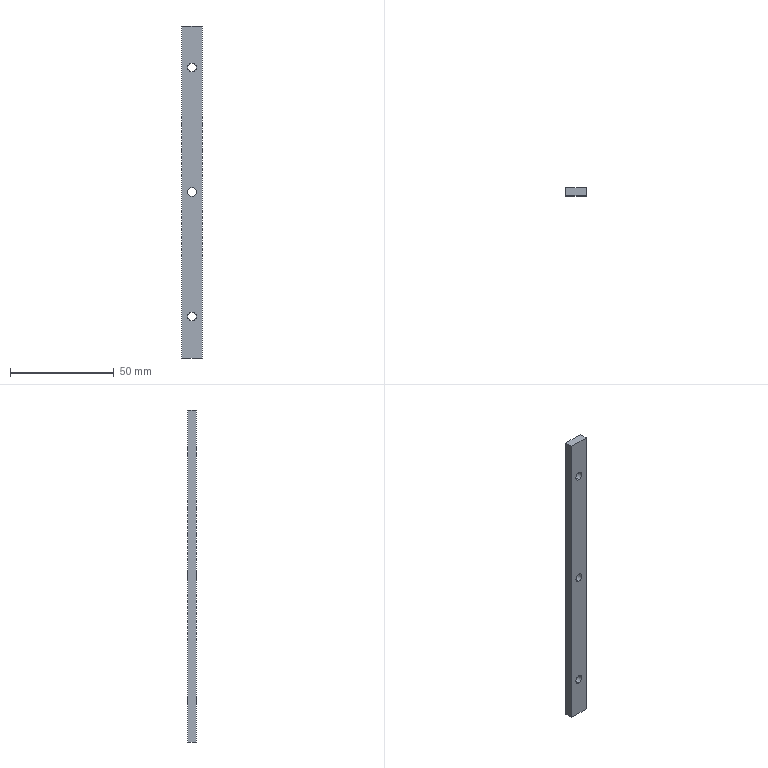Component | SolidWorks | Cover1-6XG1-1 | 1 solid | 12 faces | box 10 x 4 x 160 mm | volume 6234 mm3 | cylinder 6 | plane 6 | commonest cylinder face diameters 4.2 x6
build123d program:
from build123d import *

# Parameters (mm, degrees)
SKETCH1_W           = 160
SKETCH1_H           = 10
BOSS_EXTRUDE1_DEPTH = 4
M5_TAPPED_HOLE1_D   = 4.2


with BuildPart() as part:
    # Sketch1 → Boss-Extrude1 (new body)
    with BuildSketch(Plane.XY):
        Rectangle(SKETCH1_W, SKETCH1_H)
    extrude(amount=BOSS_EXTRUDE1_DEPTH)

    # M5 Tapped Hole1 (through all)
    with Locations(Plane.XY.offset(4)):
        with Locations((-60, 0), (0, 0), (60, 0)):
            Hole(M5_TAPPED_HOLE1_D / 2)


solid = part.part

# Placed as in the assembly
solid = solid.moved(Location((93.5, -154.8, 130), (90, 0, 90)))
STEP:
#1=CARTESIAN_POINT('',(3.681,-6.094,7.563));
#2=VERTEX_POINT('',#1);
#3=CARTESIAN_POINT('',(3.681,-6.094,7.398));
#4=VERTEX_POINT('',#3);
#5=CARTESIAN_POINT('',(3.681,-6.094,7.48));
#6=DIRECTION('',(0.,-1.,0.));
#7=DIRECTION('',(0.,0.,-1.));
#8=AXIS2_PLACEMENT_3D('',#5,#6,#7);
#9=CIRCLE('',#8,0.08268);
#10=EDGE_CURVE('',#2,#4,#9,.T.);
#11=ORIENTED_EDGE('',*,*,#10,.F.);
#12=CARTESIAN_POINT('',(3.681,-6.252,7.563));
#13=VERTEX_POINT('',#12);
#14=CARTESIAN_POINT('',(3.681,-6.252,7.563));
#15=DIRECTION('',(0.,-1.,0.));
#16=VECTOR('',#15,39.37);
#17=LINE('',#14,#16);
#18=EDGE_CURVE('',#2,#13,#17,.T.);
#19=ORIENTED_EDGE('',*,*,#18,.T.);
#20=CARTESIAN_POINT('',(3.681,-6.252,7.398));
#21=VERTEX_POINT('',#20);
#22=CARTESIAN_POINT('',(3.681,-6.252,7.48));
#23=DIRECTION('',(0.,-1.,0.));
#24=DIRECTION('',(0.,0.,-1.));
#25=AXIS2_PLACEMENT_3D('',#22,#23,#24);
#26=CIRCLE('',#25,0.08268);
#27=EDGE_CURVE('',#13,#21,#26,.T.);
#28=ORIENTED_EDGE('',*,*,#27,.T.);
#29=CARTESIAN_POINT('',(3.681,-6.252,7.398));
#30=DIRECTION('',(0.,-1.,0.));
#31=VECTOR('',#30,39.37);
#32=LINE('',#29,#31);
#33=EDGE_CURVE('',#4,#21,#32,.T.);
#34=ORIENTED_EDGE('',*,*,#33,.F.);
#35=EDGE_LOOP('',(#11,#19,#28,#34));
#36=FACE_OUTER_BOUND('',#35,.T.);
#37=CARTESIAN_POINT('',(3.681,-6.252,7.48));
#38=DIRECTION('',(0.,-1.,0.));
#39=DIRECTION('',(0.,0.,-1.));
#40=AXIS2_PLACEMENT_3D('',#37,#38,#39);
#41=CYLINDRICAL_SURFACE('',#40,0.08268);
#42=ADVANCED_FACE('',(#36),#41,.F.);
#43=CARTESIAN_POINT('',(3.681,-6.094,5.201));
#44=VERTEX_POINT('',#43);
#45=CARTESIAN_POINT('',(3.681,-6.094,5.035));
#46=VERTEX_POINT('',#45);
#47=CARTESIAN_POINT('',(3.681,-6.094,5.118));
#48=DIRECTION('',(0.,-1.,0.));
#49=DIRECTION('',(0.,0.,-1.));
#50=AXIS2_PLACEMENT_3D('',#47,#48,#49);
#51=CIRCLE('',#50,0.08268);
#52=EDGE_CURVE('',#44,#46,#51,.T.);
#53=ORIENTED_EDGE('',*,*,#52,.F.);
#54=CARTESIAN_POINT('',(3.681,-6.252,5.201));
#55=VERTEX_POINT('',#54);
#56=CARTESIAN_POINT('',(3.681,-6.252,5.201));
#57=DIRECTION('',(0.,-1.,0.));
#58=VECTOR('',#57,39.37);
#59=LINE('',#56,#58);
#60=EDGE_CURVE('',#44,#55,#59,.T.);
#61=ORIENTED_EDGE('',*,*,#60,.T.);
#62=CARTESIAN_POINT('',(3.681,-6.252,5.035));
#63=VERTEX_POINT('',#62);
#64=CARTESIAN_POINT('',(3.681,-6.252,5.118));
#65=DIRECTION('',(0.,-1.,0.));
#66=DIRECTION('',(0.,0.,-1.));
#67=AXIS2_PLACEMENT_3D('',#64,#65,#66);
#68=CIRCLE('',#67,0.08268);
#69=EDGE_CURVE('',#55,#63,#68,.T.);
#70=ORIENTED_EDGE('',*,*,#69,.T.);
#71=CARTESIAN_POINT('',(3.681,-6.252,5.035));
#72=DIRECTION('',(0.,-1.,0.));
#73=VECTOR('',#72,39.37);
#74=LINE('',#71,#73);
#75=EDGE_CURVE('',#46,#63,#74,.T.);
#76=ORIENTED_EDGE('',*,*,#75,.F.);
#77=EDGE_LOOP('',(#53,#61,#70,#76));
#78=FACE_OUTER_BOUND('',#77,.T.);
#79=CARTESIAN_POINT('',(3.681,-6.252,5.118));
#80=DIRECTION('',(0.,-1.,0.));
#81=DIRECTION('',(0.,0.,-1.));
#82=AXIS2_PLACEMENT_3D('',#79,#80,#81);
#83=CYLINDRICAL_SURFACE('',#82,0.08268);
#84=ADVANCED_FACE('',(#78),#83,.F.);
#85=CARTESIAN_POINT('',(3.681,-6.094,2.839));
#86=VERTEX_POINT('',#85);
#87=CARTESIAN_POINT('',(3.681,-6.094,2.673));
#88=VERTEX_POINT('',#87);
#89=CARTESIAN_POINT('',(3.681,-6.094,2.756));
#90=DIRECTION('',(0.,-1.,0.));
#91=DIRECTION('',(0.,0.,-1.));
#92=AXIS2_PLACEMENT_3D('',#89,#90,#91);
#93=CIRCLE('',#92,0.08268);
#94=EDGE_CURVE('',#86,#88,#93,.T.);
#95=ORIENTED_EDGE('',*,*,#94,.F.);
#96=CARTESIAN_POINT('',(3.681,-6.252,2.839));
#97=VERTEX_POINT('',#96);
#98=CARTESIAN_POINT('',(3.681,-6.252,2.839));
#99=DIRECTION('',(0.,-1.,0.));
#100=VECTOR('',#99,39.37);
#101=LINE('',#98,#100);
#102=EDGE_CURVE('',#86,#97,#101,.T.);
#103=ORIENTED_EDGE('',*,*,#102,.T.);
#104=CARTESIAN_POINT('',(3.681,-6.252,2.673));
#105=VERTEX_POINT('',#104);
#106=CARTESIAN_POINT('',(3.681,-6.252,2.756));
#107=DIRECTION('',(0.,-1.,0.));
#108=DIRECTION('',(0.,0.,-1.));
#109=AXIS2_PLACEMENT_3D('',#106,#107,#108);
#110=CIRCLE('',#109,0.08268);
#111=EDGE_CURVE('',#97,#105,#110,.T.);
#112=ORIENTED_EDGE('',*,*,#111,.T.);
#113=CARTESIAN_POINT('',(3.681,-6.252,2.673));
#114=DIRECTION('',(0.,-1.,0.));
#115=VECTOR('',#114,39.37);
#116=LINE('',#113,#115);
#117=EDGE_CURVE('',#88,#105,#116,.T.);
#118=ORIENTED_EDGE('',*,*,#117,.F.);
#119=EDGE_LOOP('',(#95,#103,#112,#118));
#120=FACE_OUTER_BOUND('',#119,.T.);
#121=CARTESIAN_POINT('',(3.681,-6.252,2.756));
#122=DIRECTION('',(0.,-1.,0.));
#123=DIRECTION('',(0.,0.,-1.));
#124=AXIS2_PLACEMENT_3D('',#121,#122,#123);
#125=CYLINDRICAL_SURFACE('',#124,0.08268);
#126=ADVANCED_FACE('',(#120),#125,.F.);
#127=CARTESIAN_POINT('',(3.878,-6.094,8.268));
#128=VERTEX_POINT('',#127);
#129=CARTESIAN_POINT('',(3.484,-6.094,8.268));
#130=VERTEX_POINT('',#129);
#131=CARTESIAN_POINT('',(3.878,-6.094,8.268));
#132=DIRECTION('',(-1.,-0.,0.));
#133=VECTOR('',#132,39.37);
#134=LINE('',#131,#133);
#135=EDGE_CURVE('',#128,#130,#134,.T.);
#136=ORIENTED_EDGE('',*,*,#135,.T.);
#137=CARTESIAN_POINT('',(3.484,-6.252,8.268));
#138=VERTEX_POINT('',#137);
#139=CARTESIAN_POINT('',(3.484,-6.252,8.268));
#140=DIRECTION('',(-0.,1.,-0.));
#141=VECTOR('',#140,39.37);
#142=LINE('',#139,#141);
#143=EDGE_CURVE('',#138,#130,#142,.T.);
#144=ORIENTED_EDGE('',*,*,#143,.F.);
#145=CARTESIAN_POINT('',(3.878,-6.252,8.268));
#146=VERTEX_POINT('',#145);
#147=CARTESIAN_POINT('',(3.878,-6.252,8.268));
#148=DIRECTION('',(-1.,-0.,0.));
#149=VECTOR('',#148,39.37);
#150=LINE('',#147,#149);
#151=EDGE_CURVE('',#146,#138,#150,.T.);
#152=ORIENTED_EDGE('',*,*,#151,.F.);
#153=CARTESIAN_POINT('',(3.878,-6.252,8.268));
#154=DIRECTION('',(-0.,1.,-0.));
#155=VECTOR('',#154,39.37);
#156=LINE('',#153,#155);
#157=EDGE_CURVE('',#146,#128,#156,.T.);
#158=ORIENTED_EDGE('',*,*,#157,.T.);
#159=EDGE_LOOP('',(#136,#144,#152,#158));
#160=FACE_OUTER_BOUND('',#159,.T.);
#161=CARTESIAN_POINT('',(3.878,-6.252,8.268));
#162=DIRECTION('',(-0.,-0.,-1.));
#163=DIRECTION('',(-0.,1.,-0.));
#164=AXIS2_PLACEMENT_3D('',#161,#162,#163);
#165=PLANE('',#164);
#166=ADVANCED_FACE('',(#160),#165,.F.);
#167=CARTESIAN_POINT('',(3.484,-6.094,1.969));
#168=VERTEX_POINT('',#167);
#169=CARTESIAN_POINT('',(3.484,-6.094,8.268));
#170=DIRECTION('',(-0.,-0.,-1.));
#171=VECTOR('',#170,39.37);
#172=LINE('',#169,#171);
#173=EDGE_CURVE('',#130,#168,#172,.T.);
#174=ORIENTED_EDGE('',*,*,#173,.T.);
#175=CARTESIAN_POINT('',(3.484,-6.252,1.969));
#176=VERTEX_POINT('',#175);
#177=CARTESIAN_POINT('',(3.484,-6.252,1.969));
#178=DIRECTION('',(-0.,1.,-0.));
#179=VECTOR('',#178,39.37);
#180=LINE('',#177,#179);
#181=EDGE_CURVE('',#176,#168,#180,.T.);
#182=ORIENTED_EDGE('',*,*,#181,.F.);
#183=CARTESIAN_POINT('',(3.484,-6.252,8.268));
#184=DIRECTION('',(-0.,-0.,-1.));
#185=VECTOR('',#184,39.37);
#186=LINE('',#183,#185);
#187=EDGE_CURVE('',#138,#176,#186,.T.);
#188=ORIENTED_EDGE('',*,*,#187,.F.);
#189=ORIENTED_EDGE('',*,*,#143,.T.);
#190=EDGE_LOOP('',(#174,#182,#188,#189));
#191=FACE_OUTER_BOUND('',#190,.T.);
#192=CARTESIAN_POINT('',(3.484,-6.252,8.268));
#193=DIRECTION('',(1.,0.,-0.));
#194=DIRECTION('',(0.,-1.,0.));
#195=AXIS2_PLACEMENT_3D('',#192,#193,#194);
#196=PLANE('',#195);
#197=ADVANCED_FACE('',(#191),#196,.F.);
#198=CARTESIAN_POINT('',(3.878,-6.094,1.969));
#199=VERTEX_POINT('',#198);
#200=CARTESIAN_POINT('',(3.878,-6.094,1.969));
#201=DIRECTION('',(1.,0.,-0.));
#202=VECTOR('',#201,39.37);
#203=LINE('',#200,#202);
#204=EDGE_CURVE('',#168,#199,#203,.T.);
#205=ORIENTED_EDGE('',*,*,#204,.T.);
#206=CARTESIAN_POINT('',(3.878,-6.252,1.969));
#207=VERTEX_POINT('',#206);
#208=CARTESIAN_POINT('',(3.878,-6.252,1.969));
#209=DIRECTION('',(-0.,1.,-0.));
#210=VECTOR('',#209,39.37);
#211=LINE('',#208,#210);
#212=EDGE_CURVE('',#207,#199,#211,.T.);
#213=ORIENTED_EDGE('',*,*,#212,.F.);
#214=CARTESIAN_POINT('',(3.878,-6.252,1.969));
#215=DIRECTION('',(1.,0.,-0.));
#216=VECTOR('',#215,39.37);
#217=LINE('',#214,#216);
#218=EDGE_CURVE('',#176,#207,#217,.T.);
#219=ORIENTED_EDGE('',*,*,#218,.F.);
#220=ORIENTED_EDGE('',*,*,#181,.T.);
#221=EDGE_LOOP('',(#205,#213,#219,#220));
#222=FACE_OUTER_BOUND('',#221,.T.);
#223=CARTESIAN_POINT('',(3.878,-6.252,1.969));
#224=DIRECTION('',(0.,0.,1.));
#225=DIRECTION('',(0.,-1.,0.));
#226=AXIS2_PLACEMENT_3D('',#223,#224,#225);
#227=PLANE('',#226);
#228=ADVANCED_FACE('',(#222),#227,.F.);
#229=CARTESIAN_POINT('',(3.878,-6.094,8.268));
#230=DIRECTION('',(0.,0.,1.));
#231=VECTOR('',#230,39.37);
#232=LINE('',#229,#231);
#233=EDGE_CURVE('',#199,#128,#232,.T.);
#234=ORIENTED_EDGE('',*,*,#233,.T.);
#235=ORIENTED_EDGE('',*,*,#157,.F.);
#236=CARTESIAN_POINT('',(3.878,-6.252,8.268));
#237=DIRECTION('',(0.,0.,1.));
#238=VECTOR('',#237,39.37);
#239=LINE('',#236,#238);
#240=EDGE_CURVE('',#207,#146,#239,.T.);
#241=ORIENTED_EDGE('',*,*,#240,.F.);
#242=ORIENTED_EDGE('',*,*,#212,.T.);
#243=EDGE_LOOP('',(#234,#235,#241,#242));
#244=FACE_OUTER_BOUND('',#243,.T.);
#245=CARTESIAN_POINT('',(3.878,-6.252,8.268));
#246=DIRECTION('',(-1.,-0.,0.));
#247=DIRECTION('',(-0.,1.,-0.));
#248=AXIS2_PLACEMENT_3D('',#245,#246,#247);
#249=PLANE('',#248);
#250=ADVANCED_FACE('',(#244),#249,.F.);
#251=CARTESIAN_POINT('',(3.681,-6.252,7.48));
#252=DIRECTION('',(0.,-1.,0.));
#253=DIRECTION('',(0.,0.,-1.));
#254=AXIS2_PLACEMENT_3D('',#251,#252,#253);
#255=CIRCLE('',#254,0.08268);
#256=EDGE_CURVE('',#21,#13,#255,.T.);
#257=ORIENTED_EDGE('',*,*,#256,.F.);
#258=ORIENTED_EDGE('',*,*,#27,.F.);
#259=EDGE_LOOP('',(#257,#258));
#260=FACE_BOUND('',#259,.T.);
#261=CARTESIAN_POINT('',(3.681,-6.252,5.118));
#262=DIRECTION('',(0.,-1.,0.));
#263=DIRECTION('',(0.,0.,-1.));
#264=AXIS2_PLACEMENT_3D('',#261,#262,#263);
#265=CIRCLE('',#264,0.08268);
#266=EDGE_CURVE('',#63,#55,#265,.T.);
#267=ORIENTED_EDGE('',*,*,#266,.F.);
#268=ORIENTED_EDGE('',*,*,#69,.F.);
#269=EDGE_LOOP('',(#267,#268));
#270=FACE_BOUND('',#269,.T.);
#271=CARTESIAN_POINT('',(3.681,-6.252,2.756));
#272=DIRECTION('',(0.,-1.,0.));
#273=DIRECTION('',(0.,0.,-1.));
#274=AXIS2_PLACEMENT_3D('',#271,#272,#273);
#275=CIRCLE('',#274,0.08268);
#276=EDGE_CURVE('',#105,#97,#275,.T.);
#277=ORIENTED_EDGE('',*,*,#276,.F.);
#278=ORIENTED_EDGE('',*,*,#111,.F.);
#279=EDGE_LOOP('',(#277,#278));
#280=FACE_BOUND('',#279,.T.);
#281=ORIENTED_EDGE('',*,*,#151,.T.);
#282=ORIENTED_EDGE('',*,*,#187,.T.);
#283=ORIENTED_EDGE('',*,*,#218,.T.);
#284=ORIENTED_EDGE('',*,*,#240,.T.);
#285=EDGE_LOOP('',(#281,#282,#283,#284));
#286=FACE_OUTER_BOUND('',#285,.T.);
#287=CARTESIAN_POINT('',(3.681,-6.252,5.118));
#288=DIRECTION('',(0.,-1.,0.));
#289=DIRECTION('',(-0.,-0.,-1.));
#290=AXIS2_PLACEMENT_3D('',#287,#288,#289);
#291=PLANE('',#290);
#292=ADVANCED_FACE('',(#260,#270,#280,#286),#291,.T.);
#293=CARTESIAN_POINT('',(3.681,-6.094,7.48));
#294=DIRECTION('',(0.,-1.,0.));
#295=DIRECTION('',(0.,0.,-1.));
#296=AXIS2_PLACEMENT_3D('',#293,#294,#295);
#297=CIRCLE('',#296,0.08268);
#298=EDGE_CURVE('',#4,#2,#297,.T.);
#299=ORIENTED_EDGE('',*,*,#298,.T.);
#300=ORIENTED_EDGE('',*,*,#10,.T.);
#301=EDGE_LOOP('',(#299,#300));
#302=FACE_BOUND('',#301,.T.);
#303=CARTESIAN_POINT('',(3.681,-6.094,5.118));
#304=DIRECTION('',(0.,-1.,0.));
#305=DIRECTION('',(0.,0.,-1.));
#306=AXIS2_PLACEMENT_3D('',#303,#304,#305);
#307=CIRCLE('',#306,0.08268);
#308=EDGE_CURVE('',#46,#44,#307,.T.);
#309=ORIENTED_EDGE('',*,*,#308,.T.);
#310=ORIENTED_EDGE('',*,*,#52,.T.);
#311=EDGE_LOOP('',(#309,#310));
#312=FACE_BOUND('',#311,.T.);
#313=CARTESIAN_POINT('',(3.681,-6.094,2.756));
#314=DIRECTION('',(0.,-1.,0.));
#315=DIRECTION('',(0.,0.,-1.));
#316=AXIS2_PLACEMENT_3D('',#313,#314,#315);
#317=CIRCLE('',#316,0.08268);
#318=EDGE_CURVE('',#88,#86,#317,.T.);
#319=ORIENTED_EDGE('',*,*,#318,.T.);
#320=ORIENTED_EDGE('',*,*,#94,.T.);
#321=EDGE_LOOP('',(#319,#320));
#322=FACE_BOUND('',#321,.T.);
#323=ORIENTED_EDGE('',*,*,#135,.F.);
#324=ORIENTED_EDGE('',*,*,#233,.F.);
#325=ORIENTED_EDGE('',*,*,#204,.F.);
#326=ORIENTED_EDGE('',*,*,#173,.F.);
#327=EDGE_LOOP('',(#323,#324,#325,#326));
#328=FACE_OUTER_BOUND('',#327,.T.);
#329=CARTESIAN_POINT('',(3.681,-6.094,5.118));
#330=DIRECTION('',(0.,-1.,0.));
#331=DIRECTION('',(-0.,-0.,-1.));
#332=AXIS2_PLACEMENT_3D('',#329,#330,#331);
#333=PLANE('',#332);
#334=ADVANCED_FACE('',(#302,#312,#322,#328),#333,.F.);
#335=ORIENTED_EDGE('',*,*,#102,.F.);
#336=ORIENTED_EDGE('',*,*,#318,.F.);
#337=ORIENTED_EDGE('',*,*,#117,.T.);
#338=ORIENTED_EDGE('',*,*,#276,.T.);
#339=EDGE_LOOP('',(#335,#336,#337,#338));
#340=FACE_OUTER_BOUND('',#339,.T.);
#341=CARTESIAN_POINT('',(3.681,-6.252,2.756));
#342=DIRECTION('',(0.,-1.,0.));
#343=DIRECTION('',(0.,0.,-1.));
#344=AXIS2_PLACEMENT_3D('',#341,#342,#343);
#345=CYLINDRICAL_SURFACE('',#344,0.08268);
#346=ADVANCED_FACE('',(#340),#345,.F.);
#347=ORIENTED_EDGE('',*,*,#60,.F.);
#348=ORIENTED_EDGE('',*,*,#308,.F.);
#349=ORIENTED_EDGE('',*,*,#75,.T.);
#350=ORIENTED_EDGE('',*,*,#266,.T.);
#351=EDGE_LOOP('',(#347,#348,#349,#350));
#352=FACE_OUTER_BOUND('',#351,.T.);
#353=CARTESIAN_POINT('',(3.681,-6.252,5.118));
#354=DIRECTION('',(0.,-1.,0.));
#355=DIRECTION('',(0.,0.,-1.));
#356=AXIS2_PLACEMENT_3D('',#353,#354,#355);
#357=CYLINDRICAL_SURFACE('',#356,0.08268);
#358=ADVANCED_FACE('',(#352),#357,.F.);
#359=ORIENTED_EDGE('',*,*,#18,.F.);
#360=ORIENTED_EDGE('',*,*,#298,.F.);
#361=ORIENTED_EDGE('',*,*,#33,.T.);
#362=ORIENTED_EDGE('',*,*,#256,.T.);
#363=EDGE_LOOP('',(#359,#360,#361,#362));
#364=FACE_OUTER_BOUND('',#363,.T.);
#365=CARTESIAN_POINT('',(3.681,-6.252,7.48));
#366=DIRECTION('',(0.,-1.,0.));
#367=DIRECTION('',(0.,0.,-1.));
#368=AXIS2_PLACEMENT_3D('',#365,#366,#367);
#369=CYLINDRICAL_SURFACE('',#368,0.08268);
#370=ADVANCED_FACE('',(#364),#369,.F.);
#371=CLOSED_SHELL('',(#42,#84,#126,#166,#197,#228,#250,#292,#334,#346,#358,#370));
#372=MANIFOLD_SOLID_BREP('',#371);
#373=CARTESIAN_POINT('',(0.,0.,0.));
#374=DIRECTION('',(0.,0.,1.));
#375=DIRECTION('',(1.,0.,0.));
#376=AXIS2_PLACEMENT_3D('',#373,#374,#375);
#377=(LENGTH_UNIT()NAMED_UNIT(*)SI_UNIT($,.METRE.));
#378=LENGTH_MEASURE_WITH_UNIT(LENGTH_MEASURE(0.0254),#377);
#379=DIMENSIONAL_EXPONENTS(1.,0.,0.,0.,0.,0.,0.);
#380=(CONVERSION_BASED_UNIT('',#378)LENGTH_UNIT()NAMED_UNIT(#379));
#381=UNCERTAINTY_MEASURE_WITH_UNIT(LENGTH_MEASURE(0.00001),#380,'','');
#382=(NAMED_UNIT(*)PLANE_ANGLE_UNIT()SI_UNIT($,.RADIAN.));
#383=(NAMED_UNIT(*)SI_UNIT($,.STERADIAN.)SOLID_ANGLE_UNIT());
#384=(GEOMETRIC_REPRESENTATION_CONTEXT(3)GLOBAL_UNCERTAINTY_ASSIGNED_CONTEXT((#381))GLOBAL_UNIT_ASSIGNED_CONTEXT((#380,#382,#383))REPRESENTATION_CONTEXT('',''));
#385=ADVANCED_BREP_SHAPE_REPRESENTATION('',(#372,#376),#384);
#386=COLOUR_RGB('',0.7922,0.8196,0.9333);
#387=FILL_AREA_STYLE_COLOUR('',#386);
#388=FILL_AREA_STYLE('',(#387));
#389=SURFACE_STYLE_FILL_AREA(#388);
#390=SURFACE_SIDE_STYLE('',(#389));
#391=SURFACE_STYLE_USAGE(.BOTH.,#390);
#392=PRESENTATION_STYLE_ASSIGNMENT((#391));
#393=STYLED_ITEM('',(#392),#372);
#394=PRESENTATION_LAYER_ASSIGNMENT('','',(#393));
#395=(LENGTH_UNIT()NAMED_UNIT(*)SI_UNIT($,.METRE.));
#396=LENGTH_MEASURE_WITH_UNIT(LENGTH_MEASURE(0.0254),#395);
#397=DIMENSIONAL_EXPONENTS(1.,0.,0.,0.,0.,0.,0.);
#398=(CONVERSION_BASED_UNIT('',#396)LENGTH_UNIT()NAMED_UNIT(#397));
#399=UNCERTAINTY_MEASURE_WITH_UNIT(LENGTH_MEASURE(0.00001),#398,'','');
#400=(NAMED_UNIT(*)PLANE_ANGLE_UNIT()SI_UNIT($,.RADIAN.));
#401=(NAMED_UNIT(*)SI_UNIT($,.STERADIAN.)SOLID_ANGLE_UNIT());
#402=(GEOMETRIC_REPRESENTATION_CONTEXT(3)GLOBAL_UNCERTAINTY_ASSIGNED_CONTEXT((#399))GLOBAL_UNIT_ASSIGNED_CONTEXT((#398,#400,#401))REPRESENTATION_CONTEXT('',''));
#403=MECHANICAL_DESIGN_GEOMETRIC_PRESENTATION_REPRESENTATION('',(#393),#402);